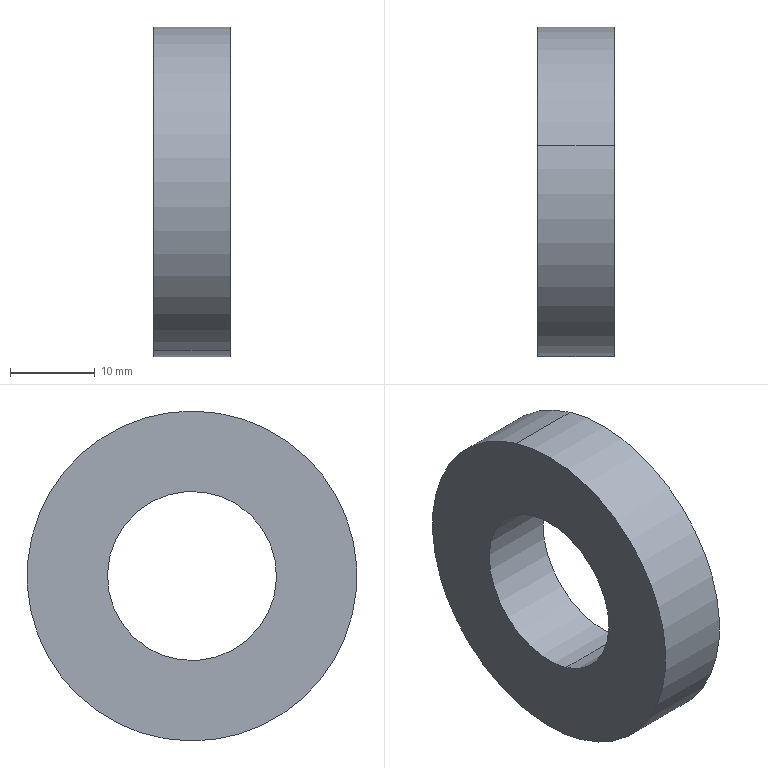Component | SolidWorks | RoundNut-1 | 1 solid | 6 faces | box 9 x 39 x 39 mm | volume 7924 mm3 | cylinder 4 | plane 2 | commonest cylinder face diameters 39 x2 20 x2
build123d program:
from build123d import *

# Parameters (mm, degrees)
SKETCH1_R           = 10
BOSS_EXTRUDE2_DEPTH = 9


with BuildPart() as part:
    # Sketch1 → Boss-Extrude2 (new body)
    with BuildSketch(Plane.XY):
        with BuildLine():
            ThreePointArc((18.025, 52.779), (7.44, 78.244), (-18.025, 67.659))
            ThreePointArc((-18.025, 67.659), (-7.44, 42.194), (18.025, 52.779))
        make_face()
        with Locations((0, 60.219)):
            Circle(SKETCH1_R, mode=Mode.SUBTRACT)
    extrude(amount=BOSS_EXTRUDE2_DEPTH)


solid = part.part

# Placed as in the assembly
solid = solid.moved(Location((-196.75, 0, 0), (0, 90, 0)))
STEP:
#1=COLOUR_RGB('',0.7922,0.8196,0.9333);
#2=FILL_AREA_STYLE_COLOUR('',#1);
#3=FILL_AREA_STYLE('',(#2));
#4=SURFACE_STYLE_FILL_AREA(#3);
#5=SURFACE_SIDE_STYLE('',(#4));
#6=SURFACE_STYLE_USAGE(.BOTH.,#5);
#7=PRESENTATION_STYLE_ASSIGNMENT((#6));
#8=CARTESIAN_POINT('',(-7.746,2.587,0.7367));
#9=VERTEX_POINT('',#8);
#10=CARTESIAN_POINT('',(-7.746,2.155,-0.7367));
#11=VERTEX_POINT('',#10);
#12=CARTESIAN_POINT('',(-7.746,2.371,0.));
#13=DIRECTION('',(-1.,0.,0.));
#14=DIRECTION('',(0.,0.2815,0.9596));
#15=AXIS2_PLACEMENT_3D('',#12,#13,#14);
#16=CIRCLE('',#15,0.7677);
#17=EDGE_CURVE('',#9,#11,#16,.T.);
#18=ORIENTED_EDGE('',*,*,#17,.F.);
#19=CARTESIAN_POINT('',(-7.392,2.587,0.7367));
#20=VERTEX_POINT('',#19);
#21=CARTESIAN_POINT('',(-7.746,2.587,0.7367));
#22=DIRECTION('',(1.,-0.,-0.));
#23=VECTOR('',#22,39.37);
#24=LINE('',#21,#23);
#25=EDGE_CURVE('',#9,#20,#24,.T.);
#26=ORIENTED_EDGE('',*,*,#25,.T.);
#27=CARTESIAN_POINT('',(-7.392,2.155,-0.7367));
#28=VERTEX_POINT('',#27);
#29=CARTESIAN_POINT('',(-7.392,2.371,0.));
#30=DIRECTION('',(-1.,0.,0.));
#31=DIRECTION('',(0.,0.2815,0.9596));
#32=AXIS2_PLACEMENT_3D('',#29,#30,#31);
#33=CIRCLE('',#32,0.7677);
#34=EDGE_CURVE('',#20,#28,#33,.T.);
#35=ORIENTED_EDGE('',*,*,#34,.T.);
#36=CARTESIAN_POINT('',(-7.746,2.155,-0.7367));
#37=DIRECTION('',(1.,-0.,-0.));
#38=VECTOR('',#37,39.37);
#39=LINE('',#36,#38);
#40=EDGE_CURVE('',#11,#28,#39,.T.);
#41=ORIENTED_EDGE('',*,*,#40,.F.);
#42=EDGE_LOOP('',(#18,#26,#35,#41));
#43=FACE_OUTER_BOUND('',#42,.T.);
#44=CARTESIAN_POINT('',(-7.746,2.371,0.));
#45=DIRECTION('',(1.,-0.,-0.));
#46=DIRECTION('',(0.,-0.2815,-0.9596));
#47=AXIS2_PLACEMENT_3D('',#44,#45,#46);
#48=CYLINDRICAL_SURFACE('',#47,0.7677);
#49=ADVANCED_FACE('',(#43),#48,.T.);
#50=CARTESIAN_POINT('',(-7.746,2.26,-0.3778));
#51=VERTEX_POINT('',#50);
#52=CARTESIAN_POINT('',(-7.746,2.482,0.3778));
#53=VERTEX_POINT('',#52);
#54=CARTESIAN_POINT('',(-7.746,2.371,0.));
#55=DIRECTION('',(-1.,0.,0.));
#56=DIRECTION('',(0.,0.2815,0.9596));
#57=AXIS2_PLACEMENT_3D('',#54,#55,#56);
#58=CIRCLE('',#57,0.3937);
#59=EDGE_CURVE('',#51,#53,#58,.T.);
#60=ORIENTED_EDGE('',*,*,#59,.T.);
#61=CARTESIAN_POINT('',(-7.392,2.482,0.3778));
#62=VERTEX_POINT('',#61);
#63=CARTESIAN_POINT('',(-7.746,2.482,0.3778));
#64=DIRECTION('',(1.,-0.,-0.));
#65=VECTOR('',#64,39.37);
#66=LINE('',#63,#65);
#67=EDGE_CURVE('',#53,#62,#66,.T.);
#68=ORIENTED_EDGE('',*,*,#67,.T.);
#69=CARTESIAN_POINT('',(-7.392,2.26,-0.3778));
#70=VERTEX_POINT('',#69);
#71=CARTESIAN_POINT('',(-7.392,2.371,0.));
#72=DIRECTION('',(-1.,0.,0.));
#73=DIRECTION('',(0.,0.2815,0.9596));
#74=AXIS2_PLACEMENT_3D('',#71,#72,#73);
#75=CIRCLE('',#74,0.3937);
#76=EDGE_CURVE('',#70,#62,#75,.T.);
#77=ORIENTED_EDGE('',*,*,#76,.F.);
#78=CARTESIAN_POINT('',(-7.746,2.26,-0.3778));
#79=DIRECTION('',(1.,-0.,-0.));
#80=VECTOR('',#79,39.37);
#81=LINE('',#78,#80);
#82=EDGE_CURVE('',#51,#70,#81,.T.);
#83=ORIENTED_EDGE('',*,*,#82,.F.);
#84=EDGE_LOOP('',(#60,#68,#77,#83));
#85=FACE_OUTER_BOUND('',#84,.T.);
#86=CARTESIAN_POINT('',(-7.746,2.371,0.));
#87=DIRECTION('',(1.,-0.,-0.));
#88=DIRECTION('',(0.,-0.2815,-0.9596));
#89=AXIS2_PLACEMENT_3D('',#86,#87,#88);
#90=CYLINDRICAL_SURFACE('',#89,0.3937);
#91=ADVANCED_FACE('',(#85),#90,.F.);
#92=ORIENTED_EDGE('',*,*,#67,.F.);
#93=CARTESIAN_POINT('',(-7.746,2.371,0.));
#94=DIRECTION('',(-1.,0.,0.));
#95=DIRECTION('',(0.,0.2815,0.9596));
#96=AXIS2_PLACEMENT_3D('',#93,#94,#95);
#97=CIRCLE('',#96,0.3937);
#98=EDGE_CURVE('',#53,#51,#97,.T.);
#99=ORIENTED_EDGE('',*,*,#98,.T.);
#100=ORIENTED_EDGE('',*,*,#82,.T.);
#101=CARTESIAN_POINT('',(-7.392,2.371,0.));
#102=DIRECTION('',(-1.,0.,0.));
#103=DIRECTION('',(0.,0.2815,0.9596));
#104=AXIS2_PLACEMENT_3D('',#101,#102,#103);
#105=CIRCLE('',#104,0.3937);
#106=EDGE_CURVE('',#62,#70,#105,.T.);
#107=ORIENTED_EDGE('',*,*,#106,.F.);
#108=EDGE_LOOP('',(#92,#99,#100,#107));
#109=FACE_OUTER_BOUND('',#108,.T.);
#110=CARTESIAN_POINT('',(-7.746,2.371,0.));
#111=DIRECTION('',(1.,-0.,-0.));
#112=DIRECTION('',(0.,-0.2815,-0.9596));
#113=AXIS2_PLACEMENT_3D('',#110,#111,#112);
#114=CYLINDRICAL_SURFACE('',#113,0.3937);
#115=ADVANCED_FACE('',(#109),#114,.F.);
#116=ORIENTED_EDGE('',*,*,#25,.F.);
#117=CARTESIAN_POINT('',(-7.746,2.371,0.));
#118=DIRECTION('',(-1.,0.,0.));
#119=DIRECTION('',(0.,0.2815,0.9596));
#120=AXIS2_PLACEMENT_3D('',#117,#118,#119);
#121=CIRCLE('',#120,0.7677);
#122=EDGE_CURVE('',#11,#9,#121,.T.);
#123=ORIENTED_EDGE('',*,*,#122,.F.);
#124=ORIENTED_EDGE('',*,*,#40,.T.);
#125=CARTESIAN_POINT('',(-7.392,2.371,0.));
#126=DIRECTION('',(-1.,0.,0.));
#127=DIRECTION('',(0.,0.2815,0.9596));
#128=AXIS2_PLACEMENT_3D('',#125,#126,#127);
#129=CIRCLE('',#128,0.7677);
#130=EDGE_CURVE('',#28,#20,#129,.T.);
#131=ORIENTED_EDGE('',*,*,#130,.T.);
#132=EDGE_LOOP('',(#116,#123,#124,#131));
#133=FACE_OUTER_BOUND('',#132,.T.);
#134=CARTESIAN_POINT('',(-7.746,2.371,0.));
#135=DIRECTION('',(1.,-0.,-0.));
#136=DIRECTION('',(0.,-0.2815,-0.9596));
#137=AXIS2_PLACEMENT_3D('',#134,#135,#136);
#138=CYLINDRICAL_SURFACE('',#137,0.7677);
#139=ADVANCED_FACE('',(#133),#138,.T.);
#140=ORIENTED_EDGE('',*,*,#59,.F.);
#141=ORIENTED_EDGE('',*,*,#98,.F.);
#142=EDGE_LOOP('',(#140,#141));
#143=FACE_BOUND('',#142,.T.);
#144=ORIENTED_EDGE('',*,*,#122,.T.);
#145=ORIENTED_EDGE('',*,*,#17,.T.);
#146=EDGE_LOOP('',(#144,#145));
#147=FACE_OUTER_BOUND('',#146,.T.);
#148=CARTESIAN_POINT('',(-7.746,0.09585,0.6673));
#149=DIRECTION('',(-1.,0.,0.));
#150=DIRECTION('',(0.,0.2815,0.9596));
#151=AXIS2_PLACEMENT_3D('',#148,#149,#150);
#152=PLANE('',#151);
#153=ADVANCED_FACE('',(#143,#147),#152,.T.);
#154=ORIENTED_EDGE('',*,*,#76,.T.);
#155=ORIENTED_EDGE('',*,*,#106,.T.);
#156=EDGE_LOOP('',(#154,#155));
#157=FACE_BOUND('',#156,.T.);
#158=ORIENTED_EDGE('',*,*,#130,.F.);
#159=ORIENTED_EDGE('',*,*,#34,.F.);
#160=EDGE_LOOP('',(#158,#159));
#161=FACE_OUTER_BOUND('',#160,.T.);
#162=CARTESIAN_POINT('',(-7.392,0.09585,0.6673));
#163=DIRECTION('',(-1.,0.,0.));
#164=DIRECTION('',(0.,0.2815,0.9596));
#165=AXIS2_PLACEMENT_3D('',#162,#163,#164);
#166=PLANE('',#165);
#167=ADVANCED_FACE('',(#157,#161),#166,.F.);
#168=CLOSED_SHELL('',(#49,#91,#115,#139,#153,#167));
#169=MANIFOLD_SOLID_BREP('',#168);
#170=STYLED_ITEM('',(#7),#169);
#171=(LENGTH_UNIT()NAMED_UNIT(*)SI_UNIT($,.METRE.));
#172=LENGTH_MEASURE_WITH_UNIT(LENGTH_MEASURE(0.0254),#171);
#173=DIMENSIONAL_EXPONENTS(1.,0.,0.,0.,0.,0.,0.);
#174=(CONVERSION_BASED_UNIT('',#172)LENGTH_UNIT()NAMED_UNIT(#173));
#175=UNCERTAINTY_MEASURE_WITH_UNIT(LENGTH_MEASURE(0.00001),#174,'','');
#176=(NAMED_UNIT(*)PLANE_ANGLE_UNIT()SI_UNIT($,.RADIAN.));
#177=(NAMED_UNIT(*)SI_UNIT($,.STERADIAN.)SOLID_ANGLE_UNIT());
#178=(GEOMETRIC_REPRESENTATION_CONTEXT(3)GLOBAL_UNCERTAINTY_ASSIGNED_CONTEXT((#175))GLOBAL_UNIT_ASSIGNED_CONTEXT((#174,#176,#177))REPRESENTATION_CONTEXT('',''));
#179=MECHANICAL_DESIGN_GEOMETRIC_PRESENTATION_REPRESENTATION('',(#170),#178);
#180=PRESENTATION_LAYER_ASSIGNMENT('','',(#170));
#181=CARTESIAN_POINT('',(0.,0.,0.));
#182=DIRECTION('',(0.,0.,1.));
#183=DIRECTION('',(1.,0.,0.));
#184=AXIS2_PLACEMENT_3D('',#181,#182,#183);
#185=(LENGTH_UNIT()NAMED_UNIT(*)SI_UNIT($,.METRE.));
#186=LENGTH_MEASURE_WITH_UNIT(LENGTH_MEASURE(0.0254),#185);
#187=DIMENSIONAL_EXPONENTS(1.,0.,0.,0.,0.,0.,0.);
#188=(CONVERSION_BASED_UNIT('',#186)LENGTH_UNIT()NAMED_UNIT(#187));
#189=UNCERTAINTY_MEASURE_WITH_UNIT(LENGTH_MEASURE(0.00001),#188,'','');
#190=(NAMED_UNIT(*)PLANE_ANGLE_UNIT()SI_UNIT($,.RADIAN.));
#191=(NAMED_UNIT(*)SI_UNIT($,.STERADIAN.)SOLID_ANGLE_UNIT());
#192=(GEOMETRIC_REPRESENTATION_CONTEXT(3)GLOBAL_UNCERTAINTY_ASSIGNED_CONTEXT((#189))GLOBAL_UNIT_ASSIGNED_CONTEXT((#188,#190,#191))REPRESENTATION_CONTEXT('',''));
#193=ADVANCED_BREP_SHAPE_REPRESENTATION('',(#169,#184),#192);